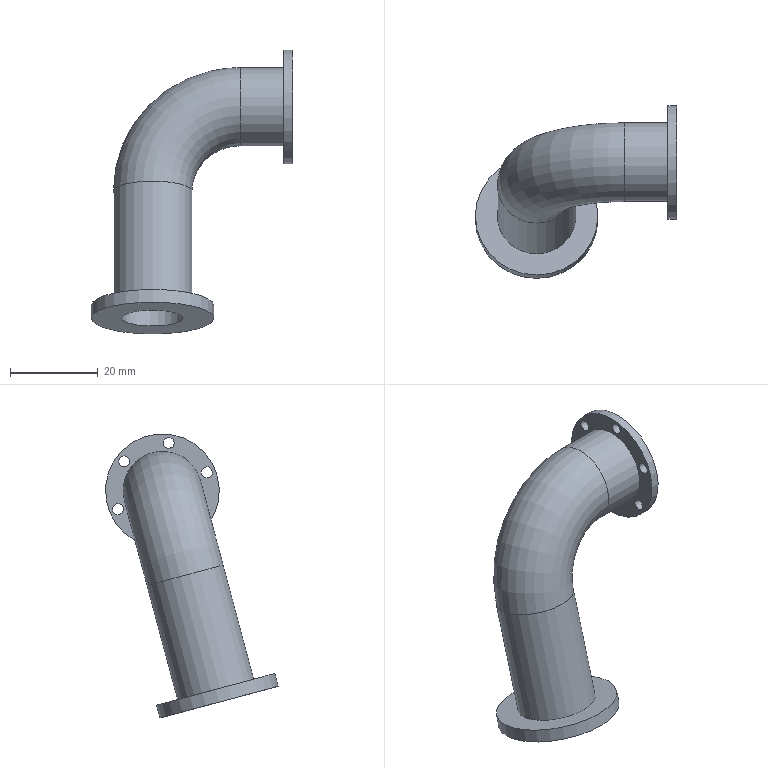Component | NX | EXT_CONN_PIPE | 1 solid | 18 faces | volume 8958 mm3 | cylinder 12 | plane 4 | torus 2 | commonest cylinder face diameters 2.5 x6 18 x2 14 x2 26 x1 28 x1